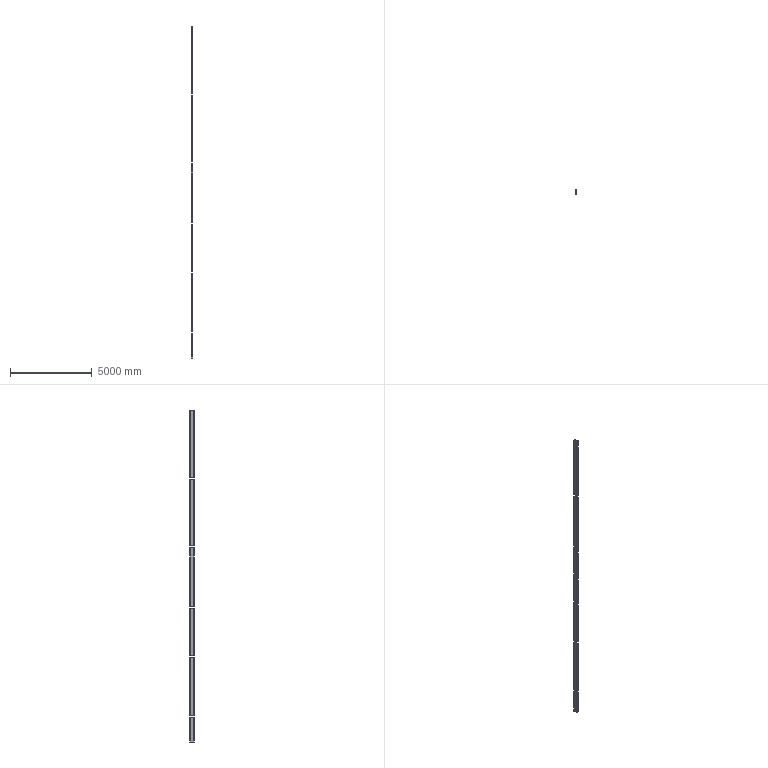Component | NX | P2_2 | 6 solids | 108 faces | volume 96349936 mm3 | plane 84 | cylinder 24 | commonest cylinder face diameters 20 x24